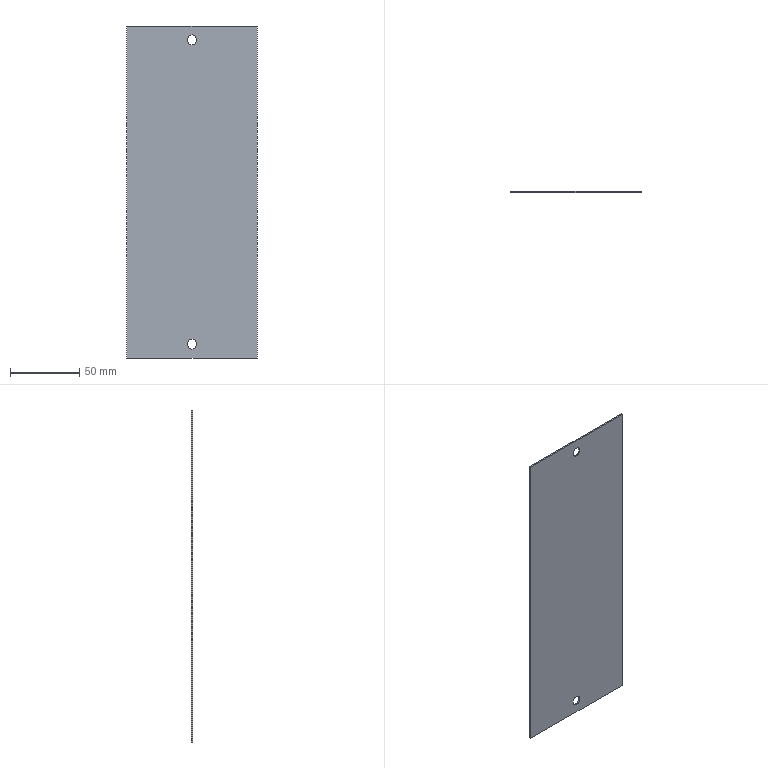Component | SolidWorks | BottomBlankingPlateCableHoleBlankingPlate2-1 | 1 solid | 10 faces | box 94 x 1 x 240 mm | volume 22483 mm3 | plane 6 | cylinder 4 | commonest cylinder face diameters 7 x4
STEP:
#1=CARTESIAN_POINT('',(8.283,-38.155,88.701));
#2=VERTEX_POINT('',#1);
#3=CARTESIAN_POINT('',(8.283,-38.155,88.977));
#4=VERTEX_POINT('',#3);
#5=CARTESIAN_POINT('',(8.283,-38.155,88.839));
#6=DIRECTION('',(0.,-1.,0.));
#7=DIRECTION('',(0.,0.,1.));
#8=AXIS2_PLACEMENT_3D('',#5,#6,#7);
#9=CIRCLE('',#8,0.1378);
#10=EDGE_CURVE('',#2,#4,#9,.T.);
#11=ORIENTED_EDGE('',*,*,#10,.F.);
#12=CARTESIAN_POINT('',(8.283,-38.194,88.701));
#13=VERTEX_POINT('',#12);
#14=CARTESIAN_POINT('',(8.283,-38.155,88.701));
#15=DIRECTION('',(0.,-1.,0.));
#16=VECTOR('',#15,39.37);
#17=LINE('',#14,#16);
#18=EDGE_CURVE('',#2,#13,#17,.T.);
#19=ORIENTED_EDGE('',*,*,#18,.T.);
#20=CARTESIAN_POINT('',(8.283,-38.194,88.977));
#21=VERTEX_POINT('',#20);
#22=CARTESIAN_POINT('',(8.283,-38.194,88.839));
#23=DIRECTION('',(0.,-1.,0.));
#24=DIRECTION('',(0.,0.,1.));
#25=AXIS2_PLACEMENT_3D('',#22,#23,#24);
#26=CIRCLE('',#25,0.1378);
#27=EDGE_CURVE('',#13,#21,#26,.T.);
#28=ORIENTED_EDGE('',*,*,#27,.T.);
#29=CARTESIAN_POINT('',(8.283,-38.155,88.977));
#30=DIRECTION('',(0.,-1.,0.));
#31=VECTOR('',#30,39.37);
#32=LINE('',#29,#31);
#33=EDGE_CURVE('',#4,#21,#32,.T.);
#34=ORIENTED_EDGE('',*,*,#33,.F.);
#35=EDGE_LOOP('',(#11,#19,#28,#34));
#36=FACE_OUTER_BOUND('',#35,.T.);
#37=CARTESIAN_POINT('',(8.283,-38.155,88.839));
#38=DIRECTION('',(0.,-1.,0.));
#39=DIRECTION('',(0.,0.,1.));
#40=AXIS2_PLACEMENT_3D('',#37,#38,#39);
#41=CYLINDRICAL_SURFACE('',#40,0.1378);
#42=ADVANCED_FACE('',(#36),#41,.F.);
#43=CARTESIAN_POINT('',(8.283,-38.155,80.04));
#44=VERTEX_POINT('',#43);
#45=CARTESIAN_POINT('',(8.283,-38.155,80.315));
#46=VERTEX_POINT('',#45);
#47=CARTESIAN_POINT('',(8.283,-38.155,80.177));
#48=DIRECTION('',(0.,-1.,0.));
#49=DIRECTION('',(0.,0.,1.));
#50=AXIS2_PLACEMENT_3D('',#47,#48,#49);
#51=CIRCLE('',#50,0.1378);
#52=EDGE_CURVE('',#44,#46,#51,.T.);
#53=ORIENTED_EDGE('',*,*,#52,.F.);
#54=CARTESIAN_POINT('',(8.283,-38.194,80.04));
#55=VERTEX_POINT('',#54);
#56=CARTESIAN_POINT('',(8.283,-38.155,80.04));
#57=DIRECTION('',(0.,-1.,0.));
#58=VECTOR('',#57,39.37);
#59=LINE('',#56,#58);
#60=EDGE_CURVE('',#44,#55,#59,.T.);
#61=ORIENTED_EDGE('',*,*,#60,.T.);
#62=CARTESIAN_POINT('',(8.283,-38.194,80.315));
#63=VERTEX_POINT('',#62);
#64=CARTESIAN_POINT('',(8.283,-38.194,80.177));
#65=DIRECTION('',(0.,-1.,0.));
#66=DIRECTION('',(0.,0.,1.));
#67=AXIS2_PLACEMENT_3D('',#64,#65,#66);
#68=CIRCLE('',#67,0.1378);
#69=EDGE_CURVE('',#55,#63,#68,.T.);
#70=ORIENTED_EDGE('',*,*,#69,.T.);
#71=CARTESIAN_POINT('',(8.283,-38.155,80.315));
#72=DIRECTION('',(0.,-1.,0.));
#73=VECTOR('',#72,39.37);
#74=LINE('',#71,#73);
#75=EDGE_CURVE('',#46,#63,#74,.T.);
#76=ORIENTED_EDGE('',*,*,#75,.F.);
#77=EDGE_LOOP('',(#53,#61,#70,#76));
#78=FACE_OUTER_BOUND('',#77,.T.);
#79=CARTESIAN_POINT('',(8.283,-38.155,80.177));
#80=DIRECTION('',(0.,-1.,0.));
#81=DIRECTION('',(0.,0.,1.));
#82=AXIS2_PLACEMENT_3D('',#79,#80,#81);
#83=CYLINDRICAL_SURFACE('',#82,0.1378);
#84=ADVANCED_FACE('',(#78),#83,.F.);
#85=CARTESIAN_POINT('',(6.432,-38.194,79.784));
#86=VERTEX_POINT('',#85);
#87=CARTESIAN_POINT('',(10.133,-38.194,79.784));
#88=VERTEX_POINT('',#87);
#89=CARTESIAN_POINT('',(10.133,-38.194,79.784));
#90=DIRECTION('',(1.,0.,-0.));
#91=VECTOR('',#90,39.37);
#92=LINE('',#89,#91);
#93=EDGE_CURVE('',#86,#88,#92,.T.);
#94=ORIENTED_EDGE('',*,*,#93,.F.);
#95=CARTESIAN_POINT('',(6.432,-38.155,79.784));
#96=VERTEX_POINT('',#95);
#97=CARTESIAN_POINT('',(6.432,-38.155,79.784));
#98=DIRECTION('',(0.,-1.,0.));
#99=VECTOR('',#98,39.37);
#100=LINE('',#97,#99);
#101=EDGE_CURVE('',#96,#86,#100,.T.);
#102=ORIENTED_EDGE('',*,*,#101,.F.);
#103=CARTESIAN_POINT('',(10.133,-38.155,79.784));
#104=VERTEX_POINT('',#103);
#105=CARTESIAN_POINT('',(10.133,-38.155,79.784));
#106=DIRECTION('',(1.,0.,-0.));
#107=VECTOR('',#106,39.37);
#108=LINE('',#105,#107);
#109=EDGE_CURVE('',#96,#104,#108,.T.);
#110=ORIENTED_EDGE('',*,*,#109,.T.);
#111=CARTESIAN_POINT('',(10.133,-38.155,79.784));
#112=DIRECTION('',(0.,-1.,0.));
#113=VECTOR('',#112,39.37);
#114=LINE('',#111,#113);
#115=EDGE_CURVE('',#104,#88,#114,.T.);
#116=ORIENTED_EDGE('',*,*,#115,.T.);
#117=EDGE_LOOP('',(#94,#102,#110,#116));
#118=FACE_OUTER_BOUND('',#117,.T.);
#119=CARTESIAN_POINT('',(10.133,-38.155,79.784));
#120=DIRECTION('',(-0.,-0.,-1.));
#121=DIRECTION('',(0.,-1.,0.));
#122=AXIS2_PLACEMENT_3D('',#119,#120,#121);
#123=PLANE('',#122);
#124=ADVANCED_FACE('',(#118),#123,.T.);
#125=CARTESIAN_POINT('',(6.432,-38.194,89.233));
#126=VERTEX_POINT('',#125);
#127=CARTESIAN_POINT('',(6.432,-38.194,79.784));
#128=DIRECTION('',(-0.,-0.,-1.));
#129=VECTOR('',#128,39.37);
#130=LINE('',#127,#129);
#131=EDGE_CURVE('',#126,#86,#130,.T.);
#132=ORIENTED_EDGE('',*,*,#131,.F.);
#133=CARTESIAN_POINT('',(6.432,-38.155,89.233));
#134=VERTEX_POINT('',#133);
#135=CARTESIAN_POINT('',(6.432,-38.155,89.233));
#136=DIRECTION('',(0.,-1.,0.));
#137=VECTOR('',#136,39.37);
#138=LINE('',#135,#137);
#139=EDGE_CURVE('',#134,#126,#138,.T.);
#140=ORIENTED_EDGE('',*,*,#139,.F.);
#141=CARTESIAN_POINT('',(6.432,-38.155,79.784));
#142=DIRECTION('',(-0.,-0.,-1.));
#143=VECTOR('',#142,39.37);
#144=LINE('',#141,#143);
#145=EDGE_CURVE('',#134,#96,#144,.T.);
#146=ORIENTED_EDGE('',*,*,#145,.T.);
#147=ORIENTED_EDGE('',*,*,#101,.T.);
#148=EDGE_LOOP('',(#132,#140,#146,#147));
#149=FACE_OUTER_BOUND('',#148,.T.);
#150=CARTESIAN_POINT('',(6.432,-38.155,79.784));
#151=DIRECTION('',(-1.,-0.,0.));
#152=DIRECTION('',(0.,-1.,0.));
#153=AXIS2_PLACEMENT_3D('',#150,#151,#152);
#154=PLANE('',#153);
#155=ADVANCED_FACE('',(#149),#154,.T.);
#156=CARTESIAN_POINT('',(10.133,-38.194,89.233));
#157=VERTEX_POINT('',#156);
#158=CARTESIAN_POINT('',(6.432,-38.194,89.233));
#159=DIRECTION('',(-1.,-0.,0.));
#160=VECTOR('',#159,39.37);
#161=LINE('',#158,#160);
#162=EDGE_CURVE('',#157,#126,#161,.T.);
#163=ORIENTED_EDGE('',*,*,#162,.F.);
#164=CARTESIAN_POINT('',(10.133,-38.155,89.233));
#165=VERTEX_POINT('',#164);
#166=CARTESIAN_POINT('',(10.133,-38.155,89.233));
#167=DIRECTION('',(0.,-1.,0.));
#168=VECTOR('',#167,39.37);
#169=LINE('',#166,#168);
#170=EDGE_CURVE('',#165,#157,#169,.T.);
#171=ORIENTED_EDGE('',*,*,#170,.F.);
#172=CARTESIAN_POINT('',(6.432,-38.155,89.233));
#173=DIRECTION('',(-1.,-0.,0.));
#174=VECTOR('',#173,39.37);
#175=LINE('',#172,#174);
#176=EDGE_CURVE('',#165,#134,#175,.T.);
#177=ORIENTED_EDGE('',*,*,#176,.T.);
#178=ORIENTED_EDGE('',*,*,#139,.T.);
#179=EDGE_LOOP('',(#163,#171,#177,#178));
#180=FACE_OUTER_BOUND('',#179,.T.);
#181=CARTESIAN_POINT('',(6.432,-38.155,89.233));
#182=DIRECTION('',(0.,0.,1.));
#183=DIRECTION('',(-0.,1.,-0.));
#184=AXIS2_PLACEMENT_3D('',#181,#182,#183);
#185=PLANE('',#184);
#186=ADVANCED_FACE('',(#180),#185,.T.);
#187=CARTESIAN_POINT('',(10.133,-38.194,89.233));
#188=DIRECTION('',(0.,0.,1.));
#189=VECTOR('',#188,39.37);
#190=LINE('',#187,#189);
#191=EDGE_CURVE('',#88,#157,#190,.T.);
#192=ORIENTED_EDGE('',*,*,#191,.F.);
#193=ORIENTED_EDGE('',*,*,#115,.F.);
#194=CARTESIAN_POINT('',(10.133,-38.155,89.233));
#195=DIRECTION('',(0.,0.,1.));
#196=VECTOR('',#195,39.37);
#197=LINE('',#194,#196);
#198=EDGE_CURVE('',#104,#165,#197,.T.);
#199=ORIENTED_EDGE('',*,*,#198,.T.);
#200=ORIENTED_EDGE('',*,*,#170,.T.);
#201=EDGE_LOOP('',(#192,#193,#199,#200));
#202=FACE_OUTER_BOUND('',#201,.T.);
#203=CARTESIAN_POINT('',(10.133,-38.155,89.233));
#204=DIRECTION('',(1.,0.,-0.));
#205=DIRECTION('',(-0.,1.,-0.));
#206=AXIS2_PLACEMENT_3D('',#203,#204,#205);
#207=PLANE('',#206);
#208=ADVANCED_FACE('',(#202),#207,.T.);
#209=CARTESIAN_POINT('',(8.283,-38.155,88.839));
#210=DIRECTION('',(0.,-1.,0.));
#211=DIRECTION('',(0.,0.,1.));
#212=AXIS2_PLACEMENT_3D('',#209,#210,#211);
#213=CIRCLE('',#212,0.1378);
#214=EDGE_CURVE('',#4,#2,#213,.T.);
#215=ORIENTED_EDGE('',*,*,#214,.T.);
#216=ORIENTED_EDGE('',*,*,#10,.T.);
#217=EDGE_LOOP('',(#215,#216));
#218=FACE_BOUND('',#217,.T.);
#219=CARTESIAN_POINT('',(8.283,-38.155,80.177));
#220=DIRECTION('',(0.,-1.,0.));
#221=DIRECTION('',(0.,0.,1.));
#222=AXIS2_PLACEMENT_3D('',#219,#220,#221);
#223=CIRCLE('',#222,0.1378);
#224=EDGE_CURVE('',#46,#44,#223,.T.);
#225=ORIENTED_EDGE('',*,*,#224,.T.);
#226=ORIENTED_EDGE('',*,*,#52,.T.);
#227=EDGE_LOOP('',(#225,#226));
#228=FACE_BOUND('',#227,.T.);
#229=ORIENTED_EDGE('',*,*,#109,.F.);
#230=ORIENTED_EDGE('',*,*,#145,.F.);
#231=ORIENTED_EDGE('',*,*,#176,.F.);
#232=ORIENTED_EDGE('',*,*,#198,.F.);
#233=EDGE_LOOP('',(#229,#230,#231,#232));
#234=FACE_OUTER_BOUND('',#233,.T.);
#235=CARTESIAN_POINT('',(291.059,-38.155,-1248.697));
#236=DIRECTION('',(-0.,1.,-0.));
#237=DIRECTION('',(-0.,-0.,-1.));
#238=AXIS2_PLACEMENT_3D('',#235,#236,#237);
#239=PLANE('',#238);
#240=ADVANCED_FACE('',(#218,#228,#234),#239,.T.);
#241=CARTESIAN_POINT('',(8.283,-38.194,88.839));
#242=DIRECTION('',(0.,-1.,0.));
#243=DIRECTION('',(0.,0.,1.));
#244=AXIS2_PLACEMENT_3D('',#241,#242,#243);
#245=CIRCLE('',#244,0.1378);
#246=EDGE_CURVE('',#21,#13,#245,.T.);
#247=ORIENTED_EDGE('',*,*,#246,.F.);
#248=ORIENTED_EDGE('',*,*,#27,.F.);
#249=EDGE_LOOP('',(#247,#248));
#250=FACE_BOUND('',#249,.T.);
#251=CARTESIAN_POINT('',(8.283,-38.194,80.177));
#252=DIRECTION('',(0.,-1.,0.));
#253=DIRECTION('',(0.,0.,1.));
#254=AXIS2_PLACEMENT_3D('',#251,#252,#253);
#255=CIRCLE('',#254,0.1378);
#256=EDGE_CURVE('',#63,#55,#255,.T.);
#257=ORIENTED_EDGE('',*,*,#256,.F.);
#258=ORIENTED_EDGE('',*,*,#69,.F.);
#259=EDGE_LOOP('',(#257,#258));
#260=FACE_BOUND('',#259,.T.);
#261=ORIENTED_EDGE('',*,*,#93,.T.);
#262=ORIENTED_EDGE('',*,*,#191,.T.);
#263=ORIENTED_EDGE('',*,*,#162,.T.);
#264=ORIENTED_EDGE('',*,*,#131,.T.);
#265=EDGE_LOOP('',(#261,#262,#263,#264));
#266=FACE_OUTER_BOUND('',#265,.T.);
#267=CARTESIAN_POINT('',(291.059,-38.194,-1248.697));
#268=DIRECTION('',(-0.,1.,-0.));
#269=DIRECTION('',(-0.,-0.,-1.));
#270=AXIS2_PLACEMENT_3D('',#267,#268,#269);
#271=PLANE('',#270);
#272=ADVANCED_FACE('',(#250,#260,#266),#271,.F.);
#273=ORIENTED_EDGE('',*,*,#60,.F.);
#274=ORIENTED_EDGE('',*,*,#224,.F.);
#275=ORIENTED_EDGE('',*,*,#75,.T.);
#276=ORIENTED_EDGE('',*,*,#256,.T.);
#277=EDGE_LOOP('',(#273,#274,#275,#276));
#278=FACE_OUTER_BOUND('',#277,.T.);
#279=CARTESIAN_POINT('',(8.283,-38.155,80.177));
#280=DIRECTION('',(0.,-1.,0.));
#281=DIRECTION('',(0.,0.,1.));
#282=AXIS2_PLACEMENT_3D('',#279,#280,#281);
#283=CYLINDRICAL_SURFACE('',#282,0.1378);
#284=ADVANCED_FACE('',(#278),#283,.F.);
#285=ORIENTED_EDGE('',*,*,#18,.F.);
#286=ORIENTED_EDGE('',*,*,#214,.F.);
#287=ORIENTED_EDGE('',*,*,#33,.T.);
#288=ORIENTED_EDGE('',*,*,#246,.T.);
#289=EDGE_LOOP('',(#285,#286,#287,#288));
#290=FACE_OUTER_BOUND('',#289,.T.);
#291=CARTESIAN_POINT('',(8.283,-38.155,88.839));
#292=DIRECTION('',(0.,-1.,0.));
#293=DIRECTION('',(0.,0.,1.));
#294=AXIS2_PLACEMENT_3D('',#291,#292,#293);
#295=CYLINDRICAL_SURFACE('',#294,0.1378);
#296=ADVANCED_FACE('',(#290),#295,.F.);
#297=CLOSED_SHELL('',(#42,#84,#124,#155,#186,#208,#240,#272,#284,#296));
#298=MANIFOLD_SOLID_BREP('',#297);
#299=CARTESIAN_POINT('',(0.,0.,0.));
#300=DIRECTION('',(0.,0.,1.));
#301=DIRECTION('',(1.,0.,0.));
#302=AXIS2_PLACEMENT_3D('',#299,#300,#301);
#303=(LENGTH_UNIT()NAMED_UNIT(*)SI_UNIT($,.METRE.));
#304=LENGTH_MEASURE_WITH_UNIT(LENGTH_MEASURE(0.0254),#303);
#305=DIMENSIONAL_EXPONENTS(1.,0.,0.,0.,0.,0.,0.);
#306=(CONVERSION_BASED_UNIT('',#304)LENGTH_UNIT()NAMED_UNIT(#305));
#307=UNCERTAINTY_MEASURE_WITH_UNIT(LENGTH_MEASURE(0.00001),#306,'','');
#308=(NAMED_UNIT(*)PLANE_ANGLE_UNIT()SI_UNIT($,.RADIAN.));
#309=(NAMED_UNIT(*)SI_UNIT($,.STERADIAN.)SOLID_ANGLE_UNIT());
#310=(GEOMETRIC_REPRESENTATION_CONTEXT(3)GLOBAL_UNCERTAINTY_ASSIGNED_CONTEXT((#307))GLOBAL_UNIT_ASSIGNED_CONTEXT((#306,#308,#309))REPRESENTATION_CONTEXT('',''));
#311=ADVANCED_BREP_SHAPE_REPRESENTATION('',(#298,#302),#310);
#312=COLOUR_RGB('',0.7922,0.8196,0.9333);
#313=FILL_AREA_STYLE_COLOUR('',#312);
#314=FILL_AREA_STYLE('',(#313));
#315=SURFACE_STYLE_FILL_AREA(#314);
#316=SURFACE_SIDE_STYLE('',(#315));
#317=SURFACE_STYLE_USAGE(.BOTH.,#316);
#318=PRESENTATION_STYLE_ASSIGNMENT((#317));
#319=STYLED_ITEM('',(#318),#298);
#320=(LENGTH_UNIT()NAMED_UNIT(*)SI_UNIT($,.METRE.));
#321=LENGTH_MEASURE_WITH_UNIT(LENGTH_MEASURE(0.0254),#320);
#322=DIMENSIONAL_EXPONENTS(1.,0.,0.,0.,0.,0.,0.);
#323=(CONVERSION_BASED_UNIT('',#321)LENGTH_UNIT()NAMED_UNIT(#322));
#324=UNCERTAINTY_MEASURE_WITH_UNIT(LENGTH_MEASURE(0.00001),#323,'','');
#325=(NAMED_UNIT(*)PLANE_ANGLE_UNIT()SI_UNIT($,.RADIAN.));
#326=(NAMED_UNIT(*)SI_UNIT($,.STERADIAN.)SOLID_ANGLE_UNIT());
#327=(GEOMETRIC_REPRESENTATION_CONTEXT(3)GLOBAL_UNCERTAINTY_ASSIGNED_CONTEXT((#324))GLOBAL_UNIT_ASSIGNED_CONTEXT((#323,#325,#326))REPRESENTATION_CONTEXT('',''));
#328=MECHANICAL_DESIGN_GEOMETRIC_PRESENTATION_REPRESENTATION('',(#319),#327);
#329=PRESENTATION_LAYER_ASSIGNMENT('','',(#319));